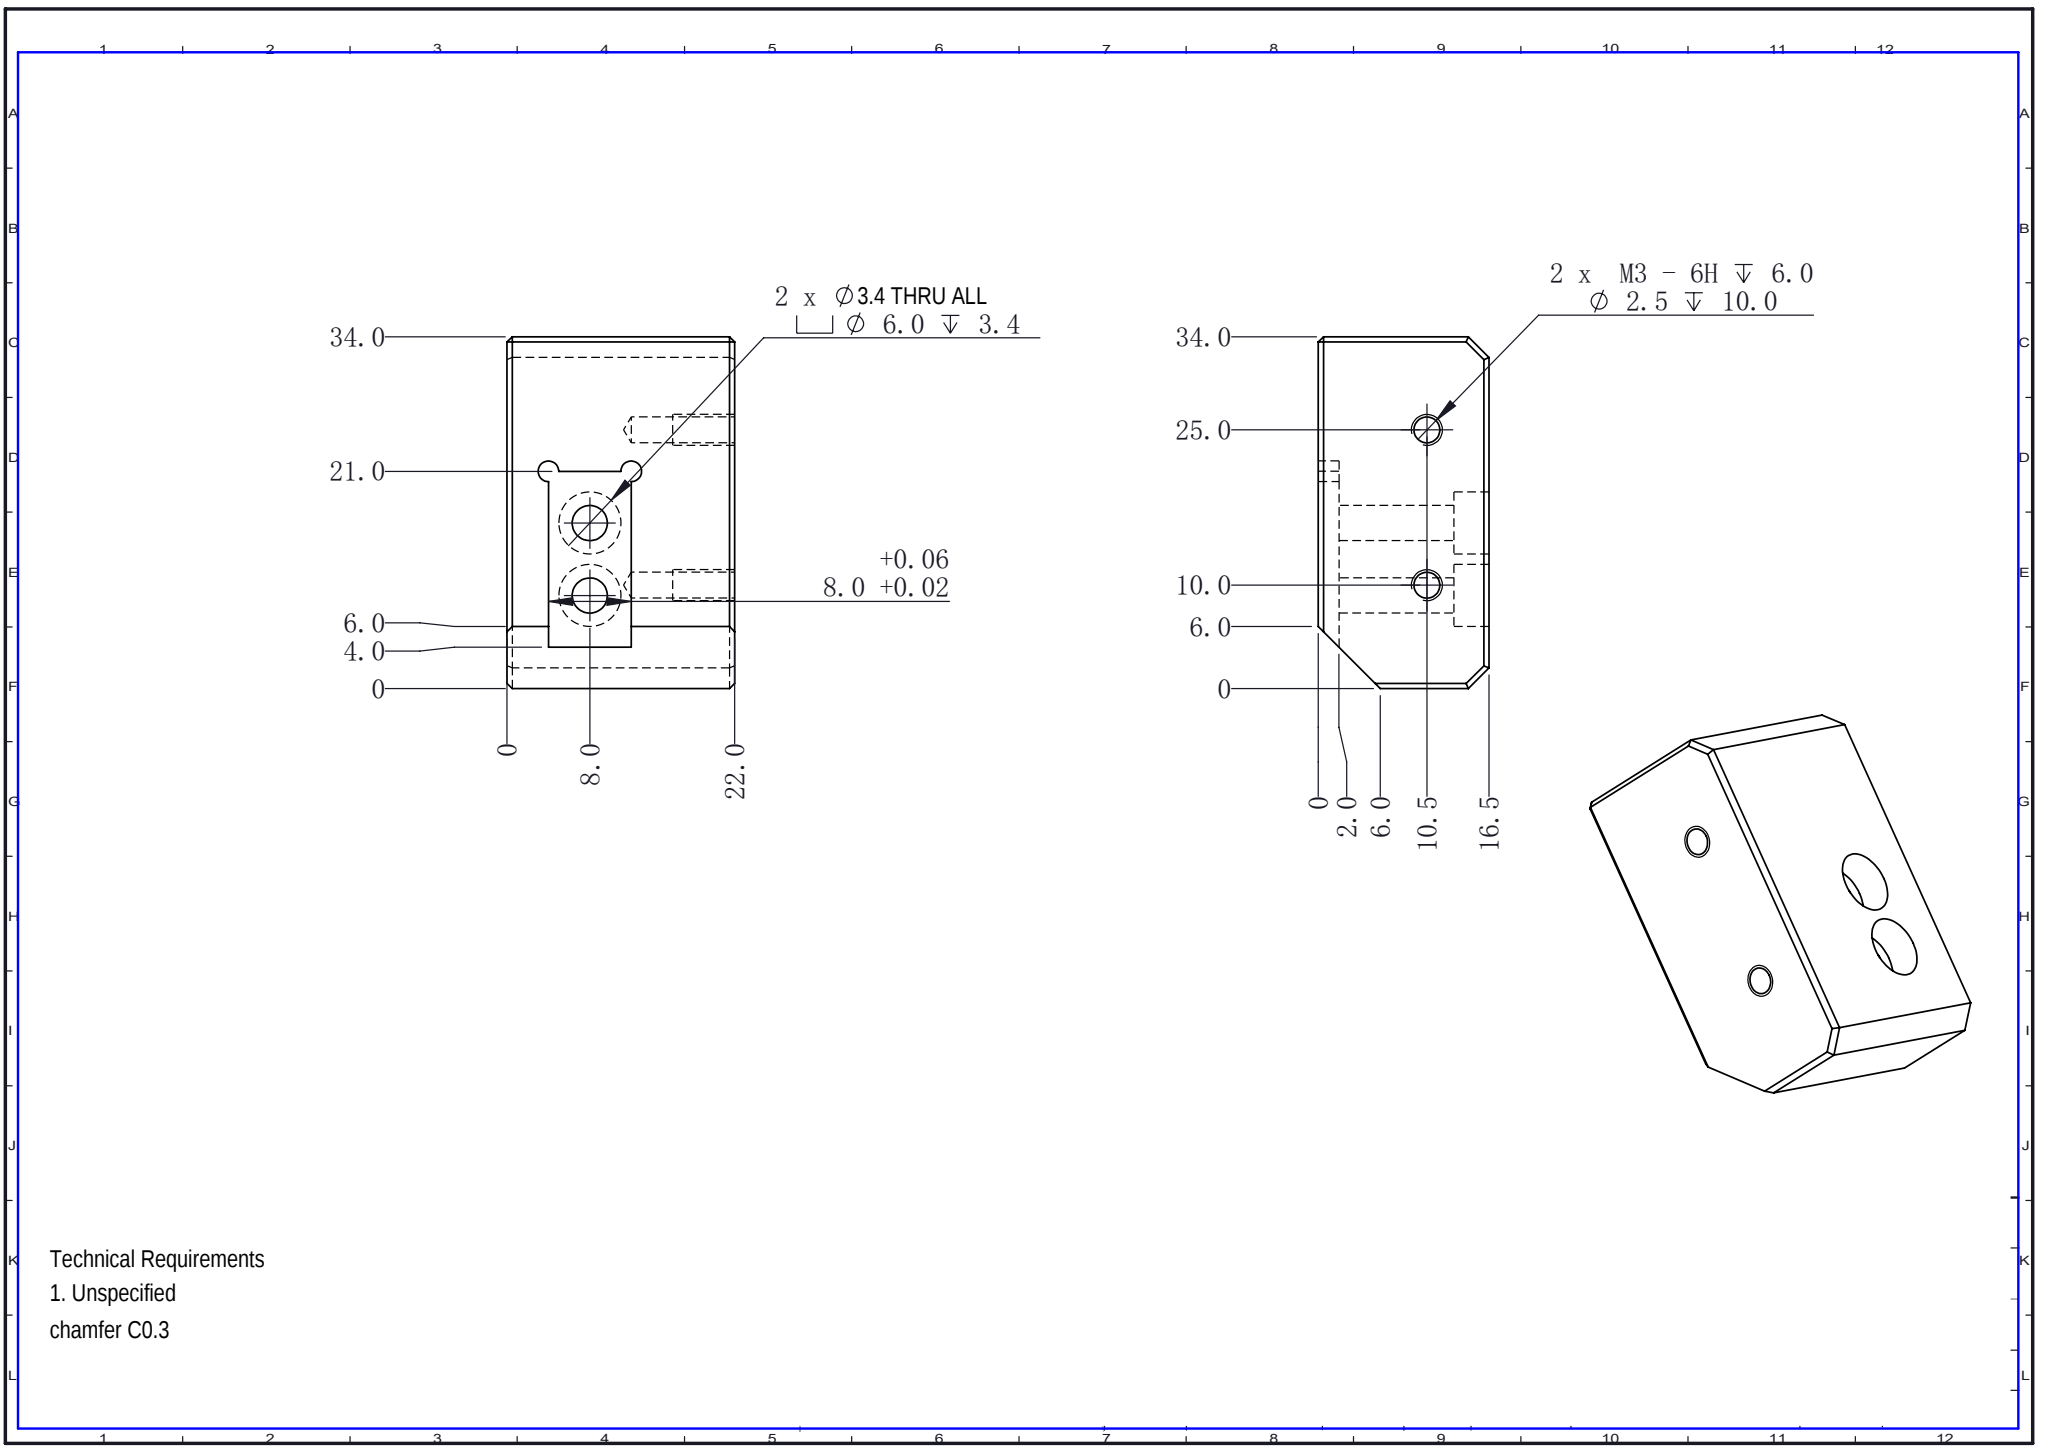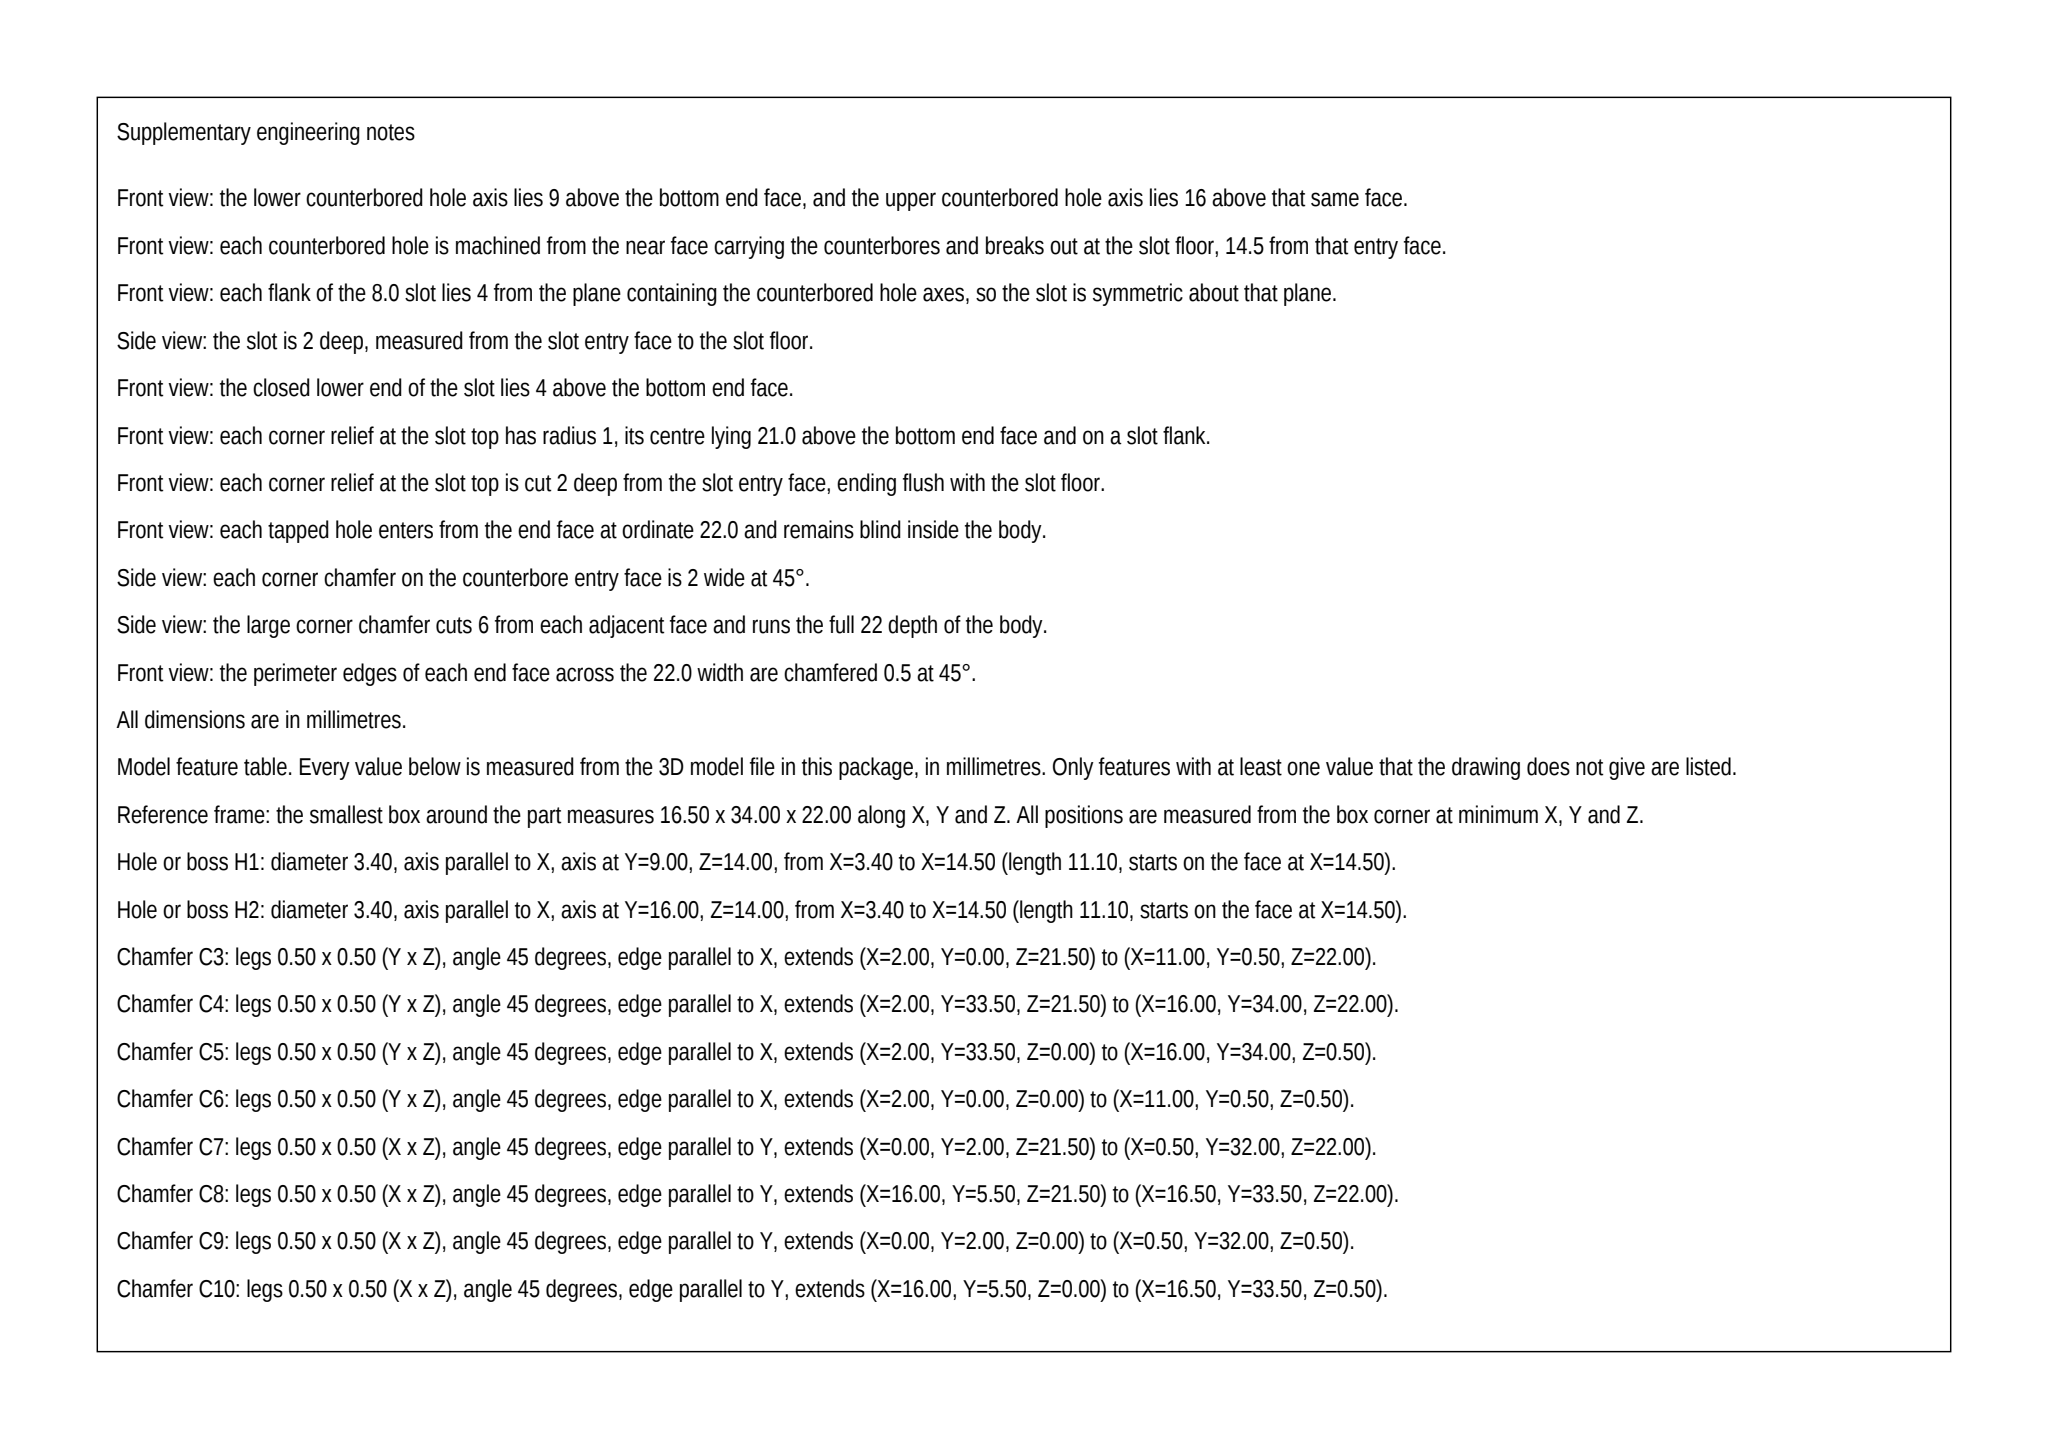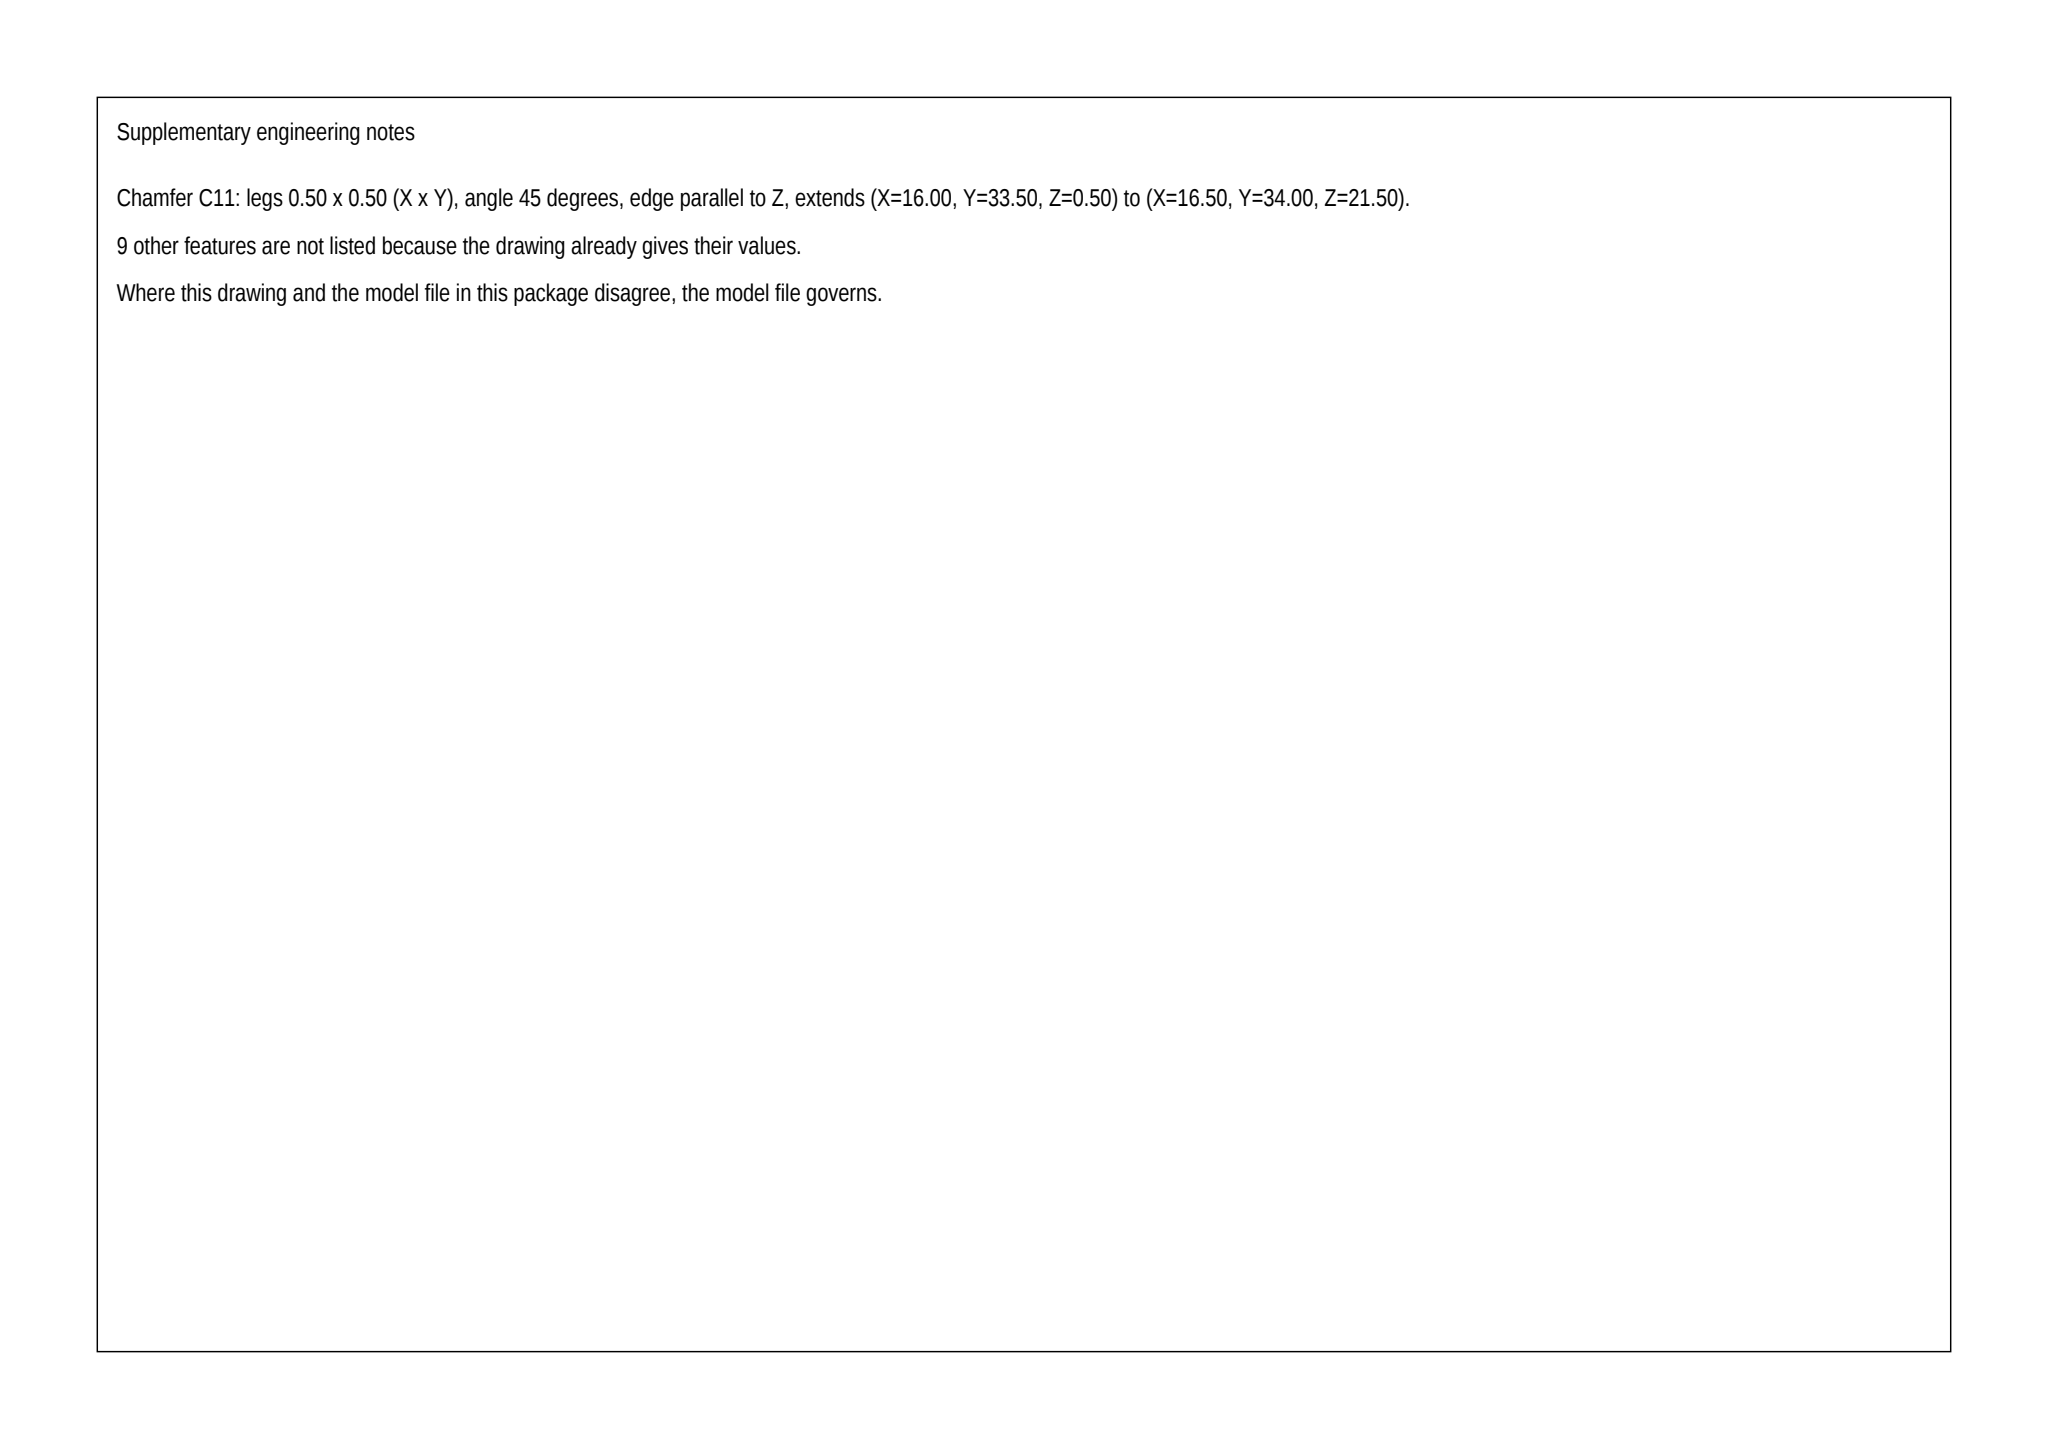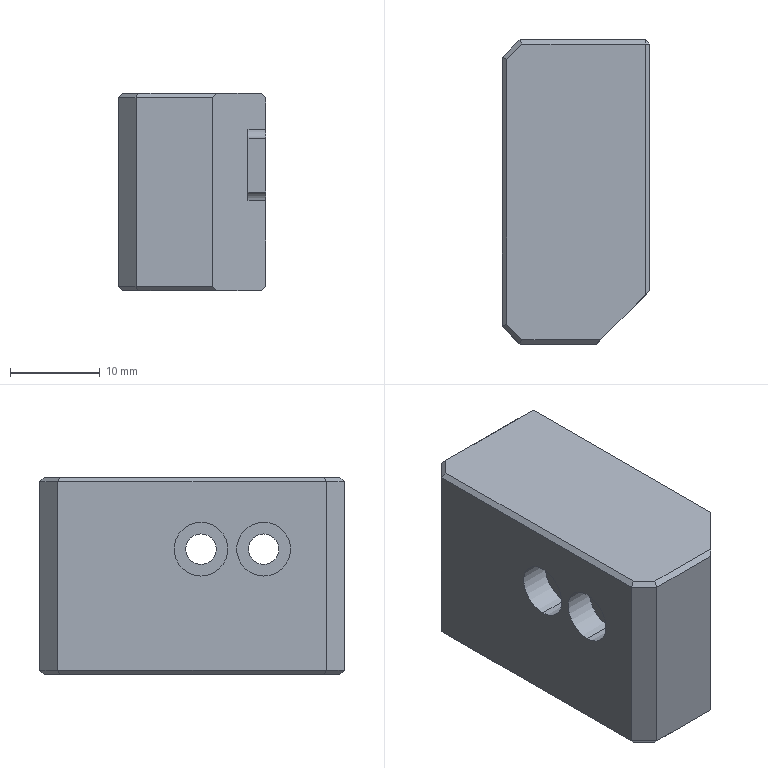Part | SolidWorks | mm | 1 solid | 49 faces | box 16.5 x 34 x 22 mm | volume 11074 mm3 | plane 30 | cylinder 15 | cone 4 | commonest cylinder face diameters 2.5 x4 6 x4 3.4 x4 2 x3
Drawing notes:
FRONT VIEW: 2X Ø3.4 C'BORE HOLE CL 9.0 & 16.0 FROM BTM (7.0 APART) | from the solid: Ø3.4 & Ø6.0 cyls, axis x, at y=9.0 and y=16.0 (bbox min corner datum = bottom face y=0)
2X Ø2.0 DP 2.0 CORNER RELIEF HOLES AT TOP OF 8.0 SLOT, CL 21.0 | from the solid: Ø2.0 cyls, axis x, length 2.0, at y=21.0, z=10.0 & 18.0 (slot walls z=10/18)